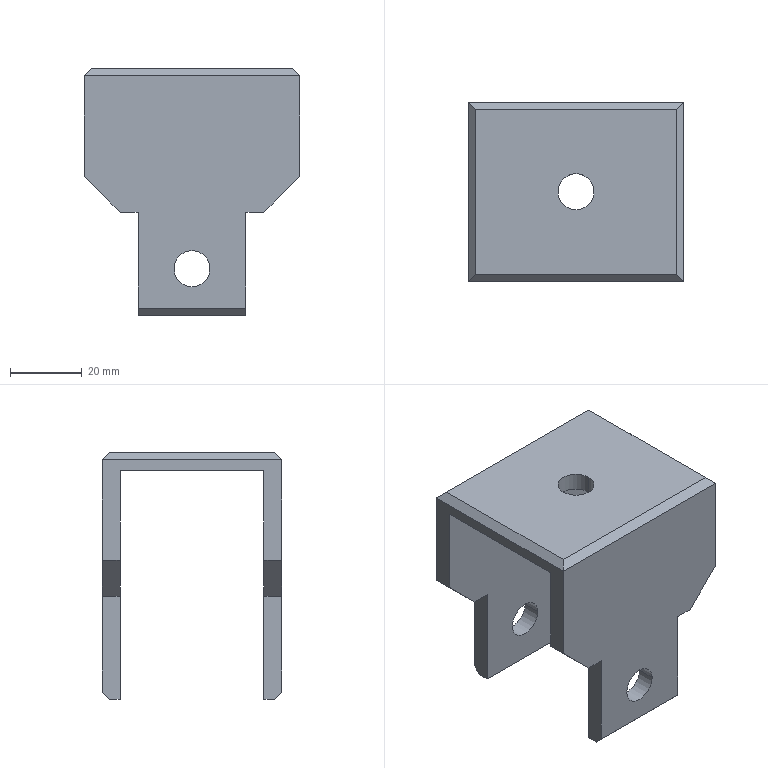Component | SolidWorks | AssemblyVibratoryFeederChassis-1_AssemblyWheel-1_WheelBracket-1 | 1 solid | 34 faces | box 60 x 50 x 68.72 mm | volume 41889 mm3 | plane 28 | cylinder 6 | commonest cylinder face diameters 10 x6
build123d program:
from build123d import *

# Parameters (mm, degrees)
EXTRUDE1_DEPTH = 60
SKETCH5_R      = 5
SKETCH5_W      = 15
SKETCH5_H      = 28.722
EXTRUDE2_DEPTH = 601.726
CHAMFER1_SIZE  = 10
SKETCH6_R      = 5
EXTRUDE3_DEPTH = 956.718
CHAMFER2_SIZE  = 2


with BuildPart() as part:
    # Sketch4 → Extrude1 (new body)
    with BuildSketch(Plane.XY):
        Polygon((-951.354, -526.906), (-901.354, -526.906), (-901.354, -595.627), (-906.354, -595.627), (-906.354, -531.906), (-946.354, -531.906), (-946.354, -595.627), (-951.354, -595.627), align=None)
    extrude(amount=-EXTRUDE1_DEPTH)

    # Sketch5 → Extrude2 (cut, through all)
    with BuildSketch(Plane.ZY.offset(951.354)):
        with Locations((-30, -582.627)):
            Circle(SKETCH5_R)
        with Locations((-52.5, -581.267)):
            Rectangle(SKETCH5_W, SKETCH5_H)
        with Locations((-7.5, -581.267)):
            Rectangle(SKETCH5_W, SKETCH5_H)
    extrude(amount=-EXTRUDE2_DEPTH, mode=Mode.SUBTRACT)

    # Chamfer1
    chamfer1_edges = [part.edges().sort_by_distance(p)[0] for p in [
        (-948.854, -566.906, -60),
        (-903.854, -566.906, -60),
        (-948.854, -566.906, 0),
        (-903.854, -566.906, 0),
    ]]
    chamfer(chamfer1_edges, length=CHAMFER1_SIZE)

    # Sketch6 → Extrude3 (cut, through all)
    with BuildSketch(Plane(origin=(0, -526.906, 0), x_dir=(1, 0, 0), z_dir=(0, 1, 0))):
        with Locations(Location((-926.354, 30, 0), (0, 0, 270))):
            Circle(SKETCH6_R)
    extrude(amount=-EXTRUDE3_DEPTH, mode=Mode.SUBTRACT)

    # Chamfer2
    chamfer2_edges = [part.edges().sort_by_distance(p)[0] for p in [
        (-951.354, -526.906, -30),
        (-901.354, -526.906, -30),
        (-926.354, -526.906, -60),
        (-951.354, -595.627, -30),
        (-901.354, -595.627, -30),
        (-926.354, -526.906, 0),
    ]]
    chamfer(chamfer2_edges, length=CHAMFER2_SIZE)


solid = part.part

# Placed as in the assembly
solid = solid.moved(Location((-307.449, -1207.53, 439.906), (90, -90, 0)))
STEP:
#1=COLOUR_RGB('',0.7922,0.8196,0.9333);
#2=FILL_AREA_STYLE_COLOUR('',#1);
#3=FILL_AREA_STYLE('',(#2));
#4=SURFACE_STYLE_FILL_AREA(#3);
#5=SURFACE_SIDE_STYLE('',(#4));
#6=SURFACE_STYLE_USAGE(.BOTH.,#5);
#7=PRESENTATION_STYLE_ASSIGNMENT((#6));
#8=CARTESIAN_POINT('',(-10.726,-11.07,-3.622));
#9=VERTEX_POINT('',#8);
#10=CARTESIAN_POINT('',(-11.12,-11.07,-3.622));
#11=VERTEX_POINT('',#10);
#12=CARTESIAN_POINT('',(-10.923,-11.07,-3.622));
#13=DIRECTION('',(-0.,-0.,-1.));
#14=DIRECTION('',(-1.,0.,0.));
#15=AXIS2_PLACEMENT_3D('',#12,#13,#14);
#16=CIRCLE('',#15,0.1969);
#17=EDGE_CURVE('',#9,#11,#16,.T.);
#18=ORIENTED_EDGE('',*,*,#17,.T.);
#19=CARTESIAN_POINT('',(-11.12,-11.07,-3.425));
#20=VERTEX_POINT('',#19);
#21=CARTESIAN_POINT('',(-11.12,-11.07,-6.131));
#22=DIRECTION('',(0.,0.,1.));
#23=VECTOR('',#22,39.37);
#24=LINE('',#21,#23);
#25=EDGE_CURVE('',#11,#20,#24,.T.);
#26=ORIENTED_EDGE('',*,*,#25,.T.);
#27=CARTESIAN_POINT('',(-10.726,-11.07,-3.425));
#28=VERTEX_POINT('',#27);
#29=CARTESIAN_POINT('',(-10.923,-11.07,-3.425));
#30=DIRECTION('',(0.,0.,1.));
#31=DIRECTION('',(1.,0.,0.));
#32=AXIS2_PLACEMENT_3D('',#29,#30,#31);
#33=CIRCLE('',#32,0.1969);
#34=EDGE_CURVE('',#20,#28,#33,.T.);
#35=ORIENTED_EDGE('',*,*,#34,.T.);
#36=CARTESIAN_POINT('',(-10.726,-11.07,-6.131));
#37=DIRECTION('',(0.,0.,1.));
#38=VECTOR('',#37,39.37);
#39=LINE('',#36,#38);
#40=EDGE_CURVE('',#9,#28,#39,.T.);
#41=ORIENTED_EDGE('',*,*,#40,.F.);
#42=EDGE_LOOP('',(#18,#26,#35,#41));
#43=FACE_OUTER_BOUND('',#42,.T.);
#44=CARTESIAN_POINT('',(-10.923,-11.07,-6.131));
#45=DIRECTION('',(0.,0.,1.));
#46=DIRECTION('',(1.,0.,0.));
#47=AXIS2_PLACEMENT_3D('',#44,#45,#46);
#48=CYLINDRICAL_SURFACE('',#47,0.1969);
#49=ADVANCED_FACE('',(#43),#48,.F.);
#50=CARTESIAN_POINT('',(-11.12,-10.086,-5.619));
#51=VERTEX_POINT('',#50);
#52=CARTESIAN_POINT('',(-10.726,-10.086,-5.619));
#53=VERTEX_POINT('',#52);
#54=CARTESIAN_POINT('',(-10.923,-10.086,-5.619));
#55=DIRECTION('',(-0.,-1.,0.));
#56=DIRECTION('',(1.,0.,0.));
#57=AXIS2_PLACEMENT_3D('',#54,#55,#56);
#58=CIRCLE('',#57,0.1969);
#59=EDGE_CURVE('',#51,#53,#58,.T.);
#60=ORIENTED_EDGE('',*,*,#59,.F.);
#61=CARTESIAN_POINT('',(-11.12,-10.283,-5.619));
#62=VERTEX_POINT('',#61);
#63=CARTESIAN_POINT('',(-11.12,-10.086,-5.619));
#64=DIRECTION('',(-0.,-1.,0.));
#65=VECTOR('',#64,39.37);
#66=LINE('',#63,#65);
#67=EDGE_CURVE('',#51,#62,#66,.T.);
#68=ORIENTED_EDGE('',*,*,#67,.T.);
#69=CARTESIAN_POINT('',(-10.726,-10.283,-5.619));
#70=VERTEX_POINT('',#69);
#71=CARTESIAN_POINT('',(-10.923,-10.283,-5.619));
#72=DIRECTION('',(-0.,-1.,0.));
#73=DIRECTION('',(1.,0.,0.));
#74=AXIS2_PLACEMENT_3D('',#71,#72,#73);
#75=CIRCLE('',#74,0.1969);
#76=EDGE_CURVE('',#62,#70,#75,.T.);
#77=ORIENTED_EDGE('',*,*,#76,.T.);
#78=CARTESIAN_POINT('',(-10.726,-10.086,-5.619));
#79=DIRECTION('',(-0.,-1.,0.));
#80=VECTOR('',#79,39.37);
#81=LINE('',#78,#80);
#82=EDGE_CURVE('',#53,#70,#81,.T.);
#83=ORIENTED_EDGE('',*,*,#82,.F.);
#84=EDGE_LOOP('',(#60,#68,#77,#83));
#85=FACE_OUTER_BOUND('',#84,.T.);
#86=CARTESIAN_POINT('',(-10.923,-10.086,-5.619));
#87=DIRECTION('',(-0.,-1.,0.));
#88=DIRECTION('',(1.,0.,0.));
#89=AXIS2_PLACEMENT_3D('',#86,#87,#88);
#90=CYLINDRICAL_SURFACE('',#89,0.1969);
#91=ADVANCED_FACE('',(#85),#90,.F.);
#92=CARTESIAN_POINT('',(-10.726,-11.857,-5.619));
#93=VERTEX_POINT('',#92);
#94=CARTESIAN_POINT('',(-11.12,-11.857,-5.619));
#95=VERTEX_POINT('',#94);
#96=CARTESIAN_POINT('',(-10.923,-11.857,-5.619));
#97=DIRECTION('',(0.,1.,-0.));
#98=DIRECTION('',(-1.,0.,0.));
#99=AXIS2_PLACEMENT_3D('',#96,#97,#98);
#100=CIRCLE('',#99,0.1969);
#101=EDGE_CURVE('',#93,#95,#100,.T.);
#102=ORIENTED_EDGE('',*,*,#101,.T.);
#103=CARTESIAN_POINT('',(-11.12,-12.054,-5.619));
#104=VERTEX_POINT('',#103);
#105=CARTESIAN_POINT('',(-11.12,-10.086,-5.619));
#106=DIRECTION('',(-0.,-1.,0.));
#107=VECTOR('',#106,39.37);
#108=LINE('',#105,#107);
#109=EDGE_CURVE('',#95,#104,#108,.T.);
#110=ORIENTED_EDGE('',*,*,#109,.T.);
#111=CARTESIAN_POINT('',(-10.726,-12.054,-5.619));
#112=VERTEX_POINT('',#111);
#113=CARTESIAN_POINT('',(-10.923,-12.054,-5.619));
#114=DIRECTION('',(-0.,-1.,0.));
#115=DIRECTION('',(1.,0.,0.));
#116=AXIS2_PLACEMENT_3D('',#113,#114,#115);
#117=CIRCLE('',#116,0.1969);
#118=EDGE_CURVE('',#104,#112,#117,.T.);
#119=ORIENTED_EDGE('',*,*,#118,.T.);
#120=CARTESIAN_POINT('',(-10.726,-10.086,-5.619));
#121=DIRECTION('',(-0.,-1.,0.));
#122=VECTOR('',#121,39.37);
#123=LINE('',#120,#122);
#124=EDGE_CURVE('',#93,#112,#123,.T.);
#125=ORIENTED_EDGE('',*,*,#124,.F.);
#126=EDGE_LOOP('',(#102,#110,#119,#125));
#127=FACE_OUTER_BOUND('',#126,.T.);
#128=CARTESIAN_POINT('',(-10.923,-10.086,-5.619));
#129=DIRECTION('',(-0.,-1.,0.));
#130=DIRECTION('',(1.,0.,0.));
#131=AXIS2_PLACEMENT_3D('',#128,#129,#130);
#132=CYLINDRICAL_SURFACE('',#131,0.1969);
#133=ADVANCED_FACE('',(#127),#132,.F.);
#134=CARTESIAN_POINT('',(-10.923,-12.054,-5.619));
#135=DIRECTION('',(-0.,-1.,0.));
#136=DIRECTION('',(1.,0.,0.));
#137=AXIS2_PLACEMENT_3D('',#134,#135,#136);
#138=CIRCLE('',#137,0.1969);
#139=EDGE_CURVE('',#112,#104,#138,.T.);
#140=ORIENTED_EDGE('',*,*,#139,.F.);
#141=ORIENTED_EDGE('',*,*,#118,.F.);
#142=EDGE_LOOP('',(#140,#141));
#143=FACE_BOUND('',#142,.T.);
#144=CARTESIAN_POINT('',(-11.514,-12.054,-6.052));
#145=VERTEX_POINT('',#144);
#146=CARTESIAN_POINT('',(-11.514,-12.054,-5.));
#147=VERTEX_POINT('',#146);
#148=CARTESIAN_POINT('',(-11.514,-12.054,-5.));
#149=DIRECTION('',(-0.,0.,1.));
#150=VECTOR('',#149,39.37);
#151=LINE('',#148,#150);
#152=EDGE_CURVE('',#145,#147,#151,.T.);
#153=ORIENTED_EDGE('',*,*,#152,.F.);
#154=CARTESIAN_POINT('',(-10.333,-12.054,-6.052));
#155=VERTEX_POINT('',#154);
#156=CARTESIAN_POINT('',(-12.104,-12.054,-6.052));
#157=DIRECTION('',(1.,-0.,-0.));
#158=VECTOR('',#157,39.37);
#159=LINE('',#156,#158);
#160=EDGE_CURVE('',#145,#155,#159,.T.);
#161=ORIENTED_EDGE('',*,*,#160,.T.);
#162=CARTESIAN_POINT('',(-10.333,-12.054,-5.));
#163=VERTEX_POINT('',#162);
#164=CARTESIAN_POINT('',(-10.333,-12.054,-5.));
#165=DIRECTION('',(-0.,-0.,-1.));
#166=VECTOR('',#165,39.37);
#167=LINE('',#164,#166);
#168=EDGE_CURVE('',#163,#155,#167,.T.);
#169=ORIENTED_EDGE('',*,*,#168,.F.);
#170=CARTESIAN_POINT('',(-10.136,-12.054,-5.));
#171=VERTEX_POINT('',#170);
#172=CARTESIAN_POINT('',(-10.333,-12.054,-5.));
#173=DIRECTION('',(-1.,0.,0.));
#174=VECTOR('',#173,39.37);
#175=LINE('',#172,#174);
#176=EDGE_CURVE('',#171,#163,#175,.T.);
#177=ORIENTED_EDGE('',*,*,#176,.F.);
#178=CARTESIAN_POINT('',(-9.742,-12.054,-4.606));
#179=VERTEX_POINT('',#178);
#180=CARTESIAN_POINT('',(-10.333,-12.054,-5.197));
#181=DIRECTION('',(0.7071,0.,0.7071));
#182=VECTOR('',#181,39.37);
#183=LINE('',#180,#182);
#184=EDGE_CURVE('',#171,#179,#183,.T.);
#185=ORIENTED_EDGE('',*,*,#184,.T.);
#186=CARTESIAN_POINT('',(-9.742,-12.054,-3.504));
#187=VERTEX_POINT('',#186);
#188=CARTESIAN_POINT('',(-9.742,-12.054,-3.425));
#189=DIRECTION('',(-0.,-0.,-1.));
#190=VECTOR('',#189,39.37);
#191=LINE('',#188,#190);
#192=EDGE_CURVE('',#187,#179,#191,.T.);
#193=ORIENTED_EDGE('',*,*,#192,.F.);
#194=CARTESIAN_POINT('',(-12.104,-12.054,-3.504));
#195=VERTEX_POINT('',#194);
#196=CARTESIAN_POINT('',(-12.104,-12.054,-3.504));
#197=DIRECTION('',(-1.,0.,0.));
#198=VECTOR('',#197,39.37);
#199=LINE('',#196,#198);
#200=EDGE_CURVE('',#187,#195,#199,.T.);
#201=ORIENTED_EDGE('',*,*,#200,.T.);
#202=CARTESIAN_POINT('',(-12.104,-12.054,-4.606));
#203=VERTEX_POINT('',#202);
#204=CARTESIAN_POINT('',(-12.104,-12.054,-3.425));
#205=DIRECTION('',(-0.,-0.,-1.));
#206=VECTOR('',#205,39.37);
#207=LINE('',#204,#206);
#208=EDGE_CURVE('',#195,#203,#207,.T.);
#209=ORIENTED_EDGE('',*,*,#208,.T.);
#210=CARTESIAN_POINT('',(-11.711,-12.054,-5.));
#211=VERTEX_POINT('',#210);
#212=CARTESIAN_POINT('',(-12.695,-12.054,-4.016));
#213=DIRECTION('',(0.7071,-0.,-0.7071));
#214=VECTOR('',#213,39.37);
#215=LINE('',#212,#214);
#216=EDGE_CURVE('',#203,#211,#215,.T.);
#217=ORIENTED_EDGE('',*,*,#216,.T.);
#218=CARTESIAN_POINT('',(-11.514,-12.054,-5.));
#219=DIRECTION('',(-1.,0.,0.));
#220=VECTOR('',#219,39.37);
#221=LINE('',#218,#220);
#222=EDGE_CURVE('',#147,#211,#221,.T.);
#223=ORIENTED_EDGE('',*,*,#222,.F.);
#224=EDGE_LOOP('',(#153,#161,#169,#177,#185,#193,#201,#209,#217,#223));
#225=FACE_OUTER_BOUND('',#224,.T.);
#226=CARTESIAN_POINT('',(-12.104,-12.054,-3.425));
#227=DIRECTION('',(-0.,-1.,0.));
#228=DIRECTION('',(1.,-0.,-0.));
#229=AXIS2_PLACEMENT_3D('',#226,#227,#228);
#230=PLANE('',#229);
#231=ADVANCED_FACE('',(#143,#225),#230,.T.);
#232=CARTESIAN_POINT('',(-9.821,-11.975,-3.425));
#233=VERTEX_POINT('',#232);
#234=CARTESIAN_POINT('',(-9.821,-10.164,-3.425));
#235=VERTEX_POINT('',#234);
#236=CARTESIAN_POINT('',(-9.821,-10.086,-3.425));
#237=DIRECTION('',(0.,1.,-0.));
#238=VECTOR('',#237,39.37);
#239=LINE('',#236,#238);
#240=EDGE_CURVE('',#233,#235,#239,.T.);
#241=ORIENTED_EDGE('',*,*,#240,.T.);
#242=CARTESIAN_POINT('',(-12.026,-10.164,-3.425));
#243=VERTEX_POINT('',#242);
#244=CARTESIAN_POINT('',(-12.104,-10.164,-3.425));
#245=DIRECTION('',(-1.,0.,0.));
#246=VECTOR('',#245,39.37);
#247=LINE('',#244,#246);
#248=EDGE_CURVE('',#235,#243,#247,.T.);
#249=ORIENTED_EDGE('',*,*,#248,.T.);
#250=CARTESIAN_POINT('',(-12.026,-11.975,-3.425));
#251=VERTEX_POINT('',#250);
#252=CARTESIAN_POINT('',(-12.026,-12.054,-3.425));
#253=DIRECTION('',(-0.,-1.,0.));
#254=VECTOR('',#253,39.37);
#255=LINE('',#252,#254);
#256=EDGE_CURVE('',#243,#251,#255,.T.);
#257=ORIENTED_EDGE('',*,*,#256,.T.);
#258=CARTESIAN_POINT('',(-12.104,-11.975,-3.425));
#259=DIRECTION('',(1.,-0.,-0.));
#260=VECTOR('',#259,39.37);
#261=LINE('',#258,#260);
#262=EDGE_CURVE('',#251,#233,#261,.T.);
#263=ORIENTED_EDGE('',*,*,#262,.T.);
#264=EDGE_LOOP('',(#241,#249,#257,#263));
#265=FACE_OUTER_BOUND('',#264,.T.);
#266=CARTESIAN_POINT('',(-10.923,-11.07,-3.425));
#267=DIRECTION('',(0.,0.,1.));
#268=DIRECTION('',(1.,0.,0.));
#269=AXIS2_PLACEMENT_3D('',#266,#267,#268);
#270=CIRCLE('',#269,0.1969);
#271=EDGE_CURVE('',#28,#20,#270,.T.);
#272=ORIENTED_EDGE('',*,*,#271,.F.);
#273=ORIENTED_EDGE('',*,*,#34,.F.);
#274=EDGE_LOOP('',(#272,#273));
#275=FACE_BOUND('',#274,.T.);
#276=CARTESIAN_POINT('',(-12.104,-12.054,-3.425));
#277=DIRECTION('',(0.,0.,1.));
#278=DIRECTION('',(1.,-0.,-0.));
#279=AXIS2_PLACEMENT_3D('',#276,#277,#278);
#280=PLANE('',#279);
#281=ADVANCED_FACE('',(#265,#275),#280,.T.);
#282=CARTESIAN_POINT('',(-10.923,-10.086,-5.619));
#283=DIRECTION('',(-0.,-1.,0.));
#284=DIRECTION('',(1.,0.,0.));
#285=AXIS2_PLACEMENT_3D('',#282,#283,#284);
#286=CIRCLE('',#285,0.1969);
#287=EDGE_CURVE('',#53,#51,#286,.T.);
#288=ORIENTED_EDGE('',*,*,#287,.T.);
#289=ORIENTED_EDGE('',*,*,#59,.T.);
#290=EDGE_LOOP('',(#288,#289));
#291=FACE_BOUND('',#290,.T.);
#292=CARTESIAN_POINT('',(-10.333,-10.086,-5.));
#293=VERTEX_POINT('',#292);
#294=CARTESIAN_POINT('',(-10.333,-10.086,-6.052));
#295=VERTEX_POINT('',#294);
#296=CARTESIAN_POINT('',(-10.333,-10.086,-5.));
#297=DIRECTION('',(-0.,-0.,-1.));
#298=VECTOR('',#297,39.37);
#299=LINE('',#296,#298);
#300=EDGE_CURVE('',#293,#295,#299,.T.);
#301=ORIENTED_EDGE('',*,*,#300,.T.);
#302=CARTESIAN_POINT('',(-11.514,-10.086,-6.052));
#303=VERTEX_POINT('',#302);
#304=CARTESIAN_POINT('',(-12.104,-10.086,-6.052));
#305=DIRECTION('',(-1.,0.,0.));
#306=VECTOR('',#305,39.37);
#307=LINE('',#304,#306);
#308=EDGE_CURVE('',#295,#303,#307,.T.);
#309=ORIENTED_EDGE('',*,*,#308,.T.);
#310=CARTESIAN_POINT('',(-11.514,-10.086,-5.));
#311=VERTEX_POINT('',#310);
#312=CARTESIAN_POINT('',(-11.514,-10.086,-5.));
#313=DIRECTION('',(-0.,0.,1.));
#314=VECTOR('',#313,39.37);
#315=LINE('',#312,#314);
#316=EDGE_CURVE('',#303,#311,#315,.T.);
#317=ORIENTED_EDGE('',*,*,#316,.T.);
#318=CARTESIAN_POINT('',(-11.711,-10.086,-5.));
#319=VERTEX_POINT('',#318);
#320=CARTESIAN_POINT('',(-11.514,-10.086,-5.));
#321=DIRECTION('',(-1.,0.,0.));
#322=VECTOR('',#321,39.37);
#323=LINE('',#320,#322);
#324=EDGE_CURVE('',#311,#319,#323,.T.);
#325=ORIENTED_EDGE('',*,*,#324,.T.);
#326=CARTESIAN_POINT('',(-12.104,-10.086,-4.606));
#327=VERTEX_POINT('',#326);
#328=CARTESIAN_POINT('',(-12.695,-10.086,-4.016));
#329=DIRECTION('',(-0.7071,0.,0.7071));
#330=VECTOR('',#329,39.37);
#331=LINE('',#328,#330);
#332=EDGE_CURVE('',#319,#327,#331,.T.);
#333=ORIENTED_EDGE('',*,*,#332,.T.);
#334=CARTESIAN_POINT('',(-12.104,-10.086,-3.504));
#335=VERTEX_POINT('',#334);
#336=CARTESIAN_POINT('',(-12.104,-10.086,-3.425));
#337=DIRECTION('',(0.,0.,1.));
#338=VECTOR('',#337,39.37);
#339=LINE('',#336,#338);
#340=EDGE_CURVE('',#327,#335,#339,.T.);
#341=ORIENTED_EDGE('',*,*,#340,.T.);
#342=CARTESIAN_POINT('',(-9.742,-10.086,-3.504));
#343=VERTEX_POINT('',#342);
#344=CARTESIAN_POINT('',(-12.104,-10.086,-3.504));
#345=DIRECTION('',(1.,-0.,-0.));
#346=VECTOR('',#345,39.37);
#347=LINE('',#344,#346);
#348=EDGE_CURVE('',#335,#343,#347,.T.);
#349=ORIENTED_EDGE('',*,*,#348,.T.);
#350=CARTESIAN_POINT('',(-9.742,-10.086,-4.606));
#351=VERTEX_POINT('',#350);
#352=CARTESIAN_POINT('',(-9.742,-10.086,-3.425));
#353=DIRECTION('',(0.,0.,1.));
#354=VECTOR('',#353,39.37);
#355=LINE('',#352,#354);
#356=EDGE_CURVE('',#351,#343,#355,.T.);
#357=ORIENTED_EDGE('',*,*,#356,.F.);
#358=CARTESIAN_POINT('',(-10.136,-10.086,-5.));
#359=VERTEX_POINT('',#358);
#360=CARTESIAN_POINT('',(-10.333,-10.086,-5.197));
#361=DIRECTION('',(-0.7071,-0.,-0.7071));
#362=VECTOR('',#361,39.37);
#363=LINE('',#360,#362);
#364=EDGE_CURVE('',#351,#359,#363,.T.);
#365=ORIENTED_EDGE('',*,*,#364,.T.);
#366=CARTESIAN_POINT('',(-10.333,-10.086,-5.));
#367=DIRECTION('',(-1.,0.,0.));
#368=VECTOR('',#367,39.37);
#369=LINE('',#366,#368);
#370=EDGE_CURVE('',#359,#293,#369,.T.);
#371=ORIENTED_EDGE('',*,*,#370,.T.);
#372=EDGE_LOOP('',(#301,#309,#317,#325,#333,#341,#349,#357,#365,#371));
#373=FACE_OUTER_BOUND('',#372,.T.);
#374=CARTESIAN_POINT('',(-12.104,-10.086,-3.425));
#375=DIRECTION('',(0.,1.,-0.));
#376=DIRECTION('',(-1.,0.,0.));
#377=AXIS2_PLACEMENT_3D('',#374,#375,#376);
#378=PLANE('',#377);
#379=ADVANCED_FACE('',(#291,#373),#378,.T.);
#380=CARTESIAN_POINT('',(-11.514,-10.164,-6.131));
#381=VERTEX_POINT('',#380);
#382=CARTESIAN_POINT('',(-11.514,-10.283,-6.131));
#383=VERTEX_POINT('',#382);
#384=CARTESIAN_POINT('',(-11.514,-10.086,-6.131));
#385=DIRECTION('',(-0.,-1.,0.));
#386=VECTOR('',#385,39.37);
#387=LINE('',#384,#386);
#388=EDGE_CURVE('',#381,#383,#387,.T.);
#389=ORIENTED_EDGE('',*,*,#388,.F.);
#390=CARTESIAN_POINT('',(-10.333,-10.164,-6.131));
#391=VERTEX_POINT('',#390);
#392=CARTESIAN_POINT('',(-12.104,-10.164,-6.131));
#393=DIRECTION('',(1.,-0.,-0.));
#394=VECTOR('',#393,39.37);
#395=LINE('',#392,#394);
#396=EDGE_CURVE('',#381,#391,#395,.T.);
#397=ORIENTED_EDGE('',*,*,#396,.T.);
#398=CARTESIAN_POINT('',(-10.333,-10.283,-6.131));
#399=VERTEX_POINT('',#398);
#400=CARTESIAN_POINT('',(-10.333,-10.086,-6.131));
#401=DIRECTION('',(-0.,-1.,0.));
#402=VECTOR('',#401,39.37);
#403=LINE('',#400,#402);
#404=EDGE_CURVE('',#391,#399,#403,.T.);
#405=ORIENTED_EDGE('',*,*,#404,.T.);
#406=CARTESIAN_POINT('',(-12.104,-10.283,-6.131));
#407=DIRECTION('',(1.,-0.,-0.));
#408=VECTOR('',#407,39.37);
#409=LINE('',#406,#408);
#410=EDGE_CURVE('',#383,#399,#409,.T.);
#411=ORIENTED_EDGE('',*,*,#410,.F.);
#412=EDGE_LOOP('',(#389,#397,#405,#411));
#413=FACE_OUTER_BOUND('',#412,.T.);
#414=CARTESIAN_POINT('',(-12.104,-10.086,-6.131));
#415=DIRECTION('',(-0.,-0.,-1.));
#416=DIRECTION('',(-1.,0.,0.));
#417=AXIS2_PLACEMENT_3D('',#414,#415,#416);
#418=PLANE('',#417);
#419=ADVANCED_FACE('',(#413),#418,.T.);
#420=CARTESIAN_POINT('',(-10.923,-10.283,-5.619));
#421=DIRECTION('',(-0.,-1.,0.));
#422=DIRECTION('',(1.,0.,0.));
#423=AXIS2_PLACEMENT_3D('',#420,#421,#422);
#424=CIRCLE('',#423,0.1969);
#425=EDGE_CURVE('',#70,#62,#424,.T.);
#426=ORIENTED_EDGE('',*,*,#425,.F.);
#427=ORIENTED_EDGE('',*,*,#76,.F.);
#428=EDGE_LOOP('',(#426,#427));
#429=FACE_BOUND('',#428,.T.);
#430=CARTESIAN_POINT('',(-10.136,-10.283,-5.));
#431=VERTEX_POINT('',#430);
#432=CARTESIAN_POINT('',(-10.333,-10.283,-5.));
#433=VERTEX_POINT('',#432);
#434=CARTESIAN_POINT('',(-12.104,-10.283,-5.));
#435=DIRECTION('',(-1.,0.,0.));
#436=VECTOR('',#435,39.37);
#437=LINE('',#434,#436);
#438=EDGE_CURVE('',#431,#433,#437,.T.);
#439=ORIENTED_EDGE('',*,*,#438,.F.);
#440=CARTESIAN_POINT('',(-9.742,-10.283,-4.606));
#441=VERTEX_POINT('',#440);
#442=CARTESIAN_POINT('',(-10.431,-10.283,-5.295));
#443=DIRECTION('',(0.7071,0.,0.7071));
#444=VECTOR('',#443,39.37);
#445=LINE('',#442,#444);
#446=EDGE_CURVE('',#431,#441,#445,.T.);
#447=ORIENTED_EDGE('',*,*,#446,.T.);
#448=CARTESIAN_POINT('',(-9.742,-10.283,-3.622));
#449=VERTEX_POINT('',#448);
#450=CARTESIAN_POINT('',(-9.742,-10.283,-3.622));
#451=DIRECTION('',(-0.,-0.,-1.));
#452=VECTOR('',#451,39.37);
#453=LINE('',#450,#452);
#454=EDGE_CURVE('',#449,#441,#453,.T.);
#455=ORIENTED_EDGE('',*,*,#454,.F.);
#456=CARTESIAN_POINT('',(-12.104,-10.283,-3.622));
#457=VERTEX_POINT('',#456);
#458=CARTESIAN_POINT('',(-12.104,-10.283,-3.622));
#459=DIRECTION('',(1.,-0.,-0.));
#460=VECTOR('',#459,39.37);
#461=LINE('',#458,#460);
#462=EDGE_CURVE('',#457,#449,#461,.T.);
#463=ORIENTED_EDGE('',*,*,#462,.F.);
#464=CARTESIAN_POINT('',(-12.104,-10.283,-4.606));
#465=VERTEX_POINT('',#464);
#466=CARTESIAN_POINT('',(-12.104,-10.283,-3.622));
#467=DIRECTION('',(-0.,-0.,-1.));
#468=VECTOR('',#467,39.37);
#469=LINE('',#466,#468);
#470=EDGE_CURVE('',#457,#465,#469,.T.);
#471=ORIENTED_EDGE('',*,*,#470,.T.);
#472=CARTESIAN_POINT('',(-11.711,-10.283,-5.));
#473=VERTEX_POINT('',#472);
#474=CARTESIAN_POINT('',(-12.596,-10.283,-4.114));
#475=DIRECTION('',(0.7071,-0.,-0.7071));
#476=VECTOR('',#475,39.37);
#477=LINE('',#474,#476);
#478=EDGE_CURVE('',#465,#473,#477,.T.);
#479=ORIENTED_EDGE('',*,*,#478,.T.);
#480=CARTESIAN_POINT('',(-11.514,-10.283,-5.));
#481=VERTEX_POINT('',#480);
#482=CARTESIAN_POINT('',(-12.104,-10.283,-5.));
#483=DIRECTION('',(-1.,0.,0.));
#484=VECTOR('',#483,39.37);
#485=LINE('',#482,#484);
#486=EDGE_CURVE('',#481,#473,#485,.T.);
#487=ORIENTED_EDGE('',*,*,#486,.F.);
#488=CARTESIAN_POINT('',(-11.514,-10.283,-3.622));
#489=DIRECTION('',(-0.,0.,1.));
#490=VECTOR('',#489,39.37);
#491=LINE('',#488,#490);
#492=EDGE_CURVE('',#383,#481,#491,.T.);
#493=ORIENTED_EDGE('',*,*,#492,.F.);
#494=ORIENTED_EDGE('',*,*,#410,.T.);
#495=CARTESIAN_POINT('',(-10.333,-10.283,-3.622));
#496=DIRECTION('',(-0.,-0.,-1.));
#497=VECTOR('',#496,39.37);
#498=LINE('',#495,#497);
#499=EDGE_CURVE('',#433,#399,#498,.T.);
#500=ORIENTED_EDGE('',*,*,#499,.F.);
#501=EDGE_LOOP('',(#439,#447,#455,#463,#471,#479,#487,#493,#494,#500));
#502=FACE_OUTER_BOUND('',#501,.T.);
#503=CARTESIAN_POINT('',(-12.104,-10.283,-3.622));
#504=DIRECTION('',(-0.,-1.,0.));
#505=DIRECTION('',(1.,-0.,-0.));
#506=AXIS2_PLACEMENT_3D('',#503,#504,#505);
#507=PLANE('',#506);
#508=ADVANCED_FACE('',(#429,#502),#507,.T.);
#509=ORIENTED_EDGE('',*,*,#17,.F.);
#510=CARTESIAN_POINT('',(-10.923,-11.07,-3.622));
#511=DIRECTION('',(-0.,-0.,-1.));
#512=DIRECTION('',(-1.,0.,0.));
#513=AXIS2_PLACEMENT_3D('',#510,#511,#512);
#514=CIRCLE('',#513,0.1969);
#515=EDGE_CURVE('',#11,#9,#514,.T.);
#516=ORIENTED_EDGE('',*,*,#515,.F.);
#517=EDGE_LOOP('',(#509,#516));
#518=FACE_BOUND('',#517,.T.);
#519=CARTESIAN_POINT('',(-9.742,-11.857,-3.622));
#520=VERTEX_POINT('',#519);
#521=CARTESIAN_POINT('',(-9.742,-11.857,-3.622));
#522=DIRECTION('',(0.,1.,-0.));
#523=VECTOR('',#522,39.37);
#524=LINE('',#521,#523);
#525=EDGE_CURVE('',#520,#449,#524,.T.);
#526=ORIENTED_EDGE('',*,*,#525,.F.);
#527=CARTESIAN_POINT('',(-12.104,-11.857,-3.622));
#528=VERTEX_POINT('',#527);
#529=CARTESIAN_POINT('',(-12.104,-11.857,-3.622));
#530=DIRECTION('',(1.,-0.,-0.));
#531=VECTOR('',#530,39.37);
#532=LINE('',#529,#531);
#533=EDGE_CURVE('',#528,#520,#532,.T.);
#534=ORIENTED_EDGE('',*,*,#533,.F.);
#535=CARTESIAN_POINT('',(-12.104,-11.857,-3.622));
#536=DIRECTION('',(0.,1.,-0.));
#537=VECTOR('',#536,39.37);
#538=LINE('',#535,#537);
#539=EDGE_CURVE('',#528,#457,#538,.T.);
#540=ORIENTED_EDGE('',*,*,#539,.T.);
#541=ORIENTED_EDGE('',*,*,#462,.T.);
#542=EDGE_LOOP('',(#526,#534,#540,#541));
#543=FACE_OUTER_BOUND('',#542,.T.);
#544=CARTESIAN_POINT('',(-12.104,-11.857,-3.622));
#545=DIRECTION('',(-0.,-0.,-1.));
#546=DIRECTION('',(-1.,0.,0.));
#547=AXIS2_PLACEMENT_3D('',#544,#545,#546);
#548=PLANE('',#547);
#549=ADVANCED_FACE('',(#518,#543),#548,.T.);
#550=ORIENTED_EDGE('',*,*,#101,.F.);
#551=CARTESIAN_POINT('',(-10.923,-11.857,-5.619));
#552=DIRECTION('',(0.,1.,-0.));
#553=DIRECTION('',(-1.,0.,0.));
#554=AXIS2_PLACEMENT_3D('',#551,#552,#553);
#555=CIRCLE('',#554,0.1969);
#556=EDGE_CURVE('',#95,#93,#555,.T.);
#557=ORIENTED_EDGE('',*,*,#556,.F.);
#558=EDGE_LOOP('',(#550,#557));
#559=FACE_BOUND('',#558,.T.);
#560=CARTESIAN_POINT('',(-9.742,-11.857,-4.606));
#561=VERTEX_POINT('',#560);
#562=CARTESIAN_POINT('',(-9.742,-11.857,-3.622));
#563=DIRECTION('',(0.,0.,1.));
#564=VECTOR('',#563,39.37);
#565=LINE('',#562,#564);
#566=EDGE_CURVE('',#561,#520,#565,.T.);
#567=ORIENTED_EDGE('',*,*,#566,.F.);
#568=CARTESIAN_POINT('',(-10.136,-11.857,-5.));
#569=VERTEX_POINT('',#568);
#570=CARTESIAN_POINT('',(-10.431,-11.857,-5.295));
#571=DIRECTION('',(-0.7071,-0.,-0.7071));
#572=VECTOR('',#571,39.37);
#573=LINE('',#570,#572);
#574=EDGE_CURVE('',#561,#569,#573,.T.);
#575=ORIENTED_EDGE('',*,*,#574,.T.);
#576=CARTESIAN_POINT('',(-10.333,-11.857,-5.));
#577=VERTEX_POINT('',#576);
#578=CARTESIAN_POINT('',(-12.104,-11.857,-5.));
#579=DIRECTION('',(1.,-0.,-0.));
#580=VECTOR('',#579,39.37);
#581=LINE('',#578,#580);
#582=EDGE_CURVE('',#577,#569,#581,.T.);
#583=ORIENTED_EDGE('',*,*,#582,.F.);
#584=CARTESIAN_POINT('',(-10.333,-11.857,-6.131));
#585=VERTEX_POINT('',#584);
#586=CARTESIAN_POINT('',(-10.333,-11.857,-3.622));
#587=DIRECTION('',(0.,0.,1.));
#588=VECTOR('',#587,39.37);
#589=LINE('',#586,#588);
#590=EDGE_CURVE('',#585,#577,#589,.T.);
#591=ORIENTED_EDGE('',*,*,#590,.F.);
#592=CARTESIAN_POINT('',(-11.514,-11.857,-6.131));
#593=VERTEX_POINT('',#592);
#594=CARTESIAN_POINT('',(-12.104,-11.857,-6.131));
#595=DIRECTION('',(1.,-0.,-0.));
#596=VECTOR('',#595,39.37);
#597=LINE('',#594,#596);
#598=EDGE_CURVE('',#593,#585,#597,.T.);
#599=ORIENTED_EDGE('',*,*,#598,.F.);
#600=CARTESIAN_POINT('',(-11.514,-11.857,-5.));
#601=VERTEX_POINT('',#600);
#602=CARTESIAN_POINT('',(-11.514,-11.857,-3.622));
#603=DIRECTION('',(0.,-0.,-1.));
#604=VECTOR('',#603,39.37);
#605=LINE('',#602,#604);
#606=EDGE_CURVE('',#601,#593,#605,.T.);
#607=ORIENTED_EDGE('',*,*,#606,.F.);
#608=CARTESIAN_POINT('',(-11.711,-11.857,-5.));
#609=VERTEX_POINT('',#608);
#610=CARTESIAN_POINT('',(-12.104,-11.857,-5.));
#611=DIRECTION('',(1.,-0.,-0.));
#612=VECTOR('',#611,39.37);
#613=LINE('',#610,#612);
#614=EDGE_CURVE('',#609,#601,#613,.T.);
#615=ORIENTED_EDGE('',*,*,#614,.F.);
#616=CARTESIAN_POINT('',(-12.104,-11.857,-4.606));
#617=VERTEX_POINT('',#616);
#618=CARTESIAN_POINT('',(-12.596,-11.857,-4.114));
#619=DIRECTION('',(-0.7071,0.,0.7071));
#620=VECTOR('',#619,39.37);
#621=LINE('',#618,#620);
#622=EDGE_CURVE('',#609,#617,#621,.T.);
#623=ORIENTED_EDGE('',*,*,#622,.T.);
#624=CARTESIAN_POINT('',(-12.104,-11.857,-3.622));
#625=DIRECTION('',(0.,0.,1.));
#626=VECTOR('',#625,39.37);
#627=LINE('',#624,#626);
#628=EDGE_CURVE('',#617,#528,#627,.T.);
#629=ORIENTED_EDGE('',*,*,#628,.T.);
#630=ORIENTED_EDGE('',*,*,#533,.T.);
#631=EDGE_LOOP('',(#567,#575,#583,#591,#599,#607,#615,#623,#629,#630));
#632=FACE_OUTER_BOUND('',#631,.T.);
#633=CARTESIAN_POINT('',(-12.104,-11.857,-3.622));
#634=DIRECTION('',(0.,1.,-0.));
#635=DIRECTION('',(-1.,0.,0.));
#636=AXIS2_PLACEMENT_3D('',#633,#634,#635);
#637=PLANE('',#636);
#638=ADVANCED_FACE('',(#559,#632),#637,.T.);
#639=CARTESIAN_POINT('',(-10.333,-11.975,-6.131));
#640=VERTEX_POINT('',#639);
#641=CARTESIAN_POINT('',(-10.333,-10.086,-6.131));
#642=DIRECTION('',(-0.,-1.,0.));
#643=VECTOR('',#642,39.37);
#644=LINE('',#641,#643);
#645=EDGE_CURVE('',#585,#640,#644,.T.);
#646=ORIENTED_EDGE('',*,*,#645,.T.);
#647=CARTESIAN_POINT('',(-11.514,-11.975,-6.131));
#648=VERTEX_POINT('',#647);
#649=CARTESIAN_POINT('',(-12.104,-11.975,-6.131));
#650=DIRECTION('',(-1.,0.,0.));
#651=VECTOR('',#650,39.37);
#652=LINE('',#649,#651);
#653=EDGE_CURVE('',#640,#648,#652,.T.);
#654=ORIENTED_EDGE('',*,*,#653,.T.);
#655=CARTESIAN_POINT('',(-11.514,-10.086,-6.131));
#656=DIRECTION('',(-0.,-1.,0.));
#657=VECTOR('',#656,39.37);
#658=LINE('',#655,#657);
#659=EDGE_CURVE('',#593,#648,#658,.T.);
#660=ORIENTED_EDGE('',*,*,#659,.F.);
#661=ORIENTED_EDGE('',*,*,#598,.T.);
#662=EDGE_LOOP('',(#646,#654,#660,#661));
#663=FACE_OUTER_BOUND('',#662,.T.);
#664=CARTESIAN_POINT('',(-12.104,-11.857,-6.131));
#665=DIRECTION('',(-0.,-0.,-1.));
#666=DIRECTION('',(-1.,0.,0.));
#667=AXIS2_PLACEMENT_3D('',#664,#665,#666);
#668=PLANE('',#667);
#669=ADVANCED_FACE('',(#663),#668,.T.);
#670=ORIENTED_EDGE('',*,*,#208,.F.);
#671=CARTESIAN_POINT('',(-12.104,-12.054,-3.504));
#672=DIRECTION('',(0.,1.,-0.));
#673=VECTOR('',#672,39.37);
#674=LINE('',#671,#673);
#675=EDGE_CURVE('',#195,#335,#674,.T.);
#676=ORIENTED_EDGE('',*,*,#675,.T.);
#677=ORIENTED_EDGE('',*,*,#340,.F.);
#678=CARTESIAN_POINT('',(-12.104,-10.283,-4.606));
#679=DIRECTION('',(-0.,-1.,0.));
#680=VECTOR('',#679,39.37);
#681=LINE('',#678,#680);
#682=EDGE_CURVE('',#327,#465,#681,.T.);
#683=ORIENTED_EDGE('',*,*,#682,.T.);
#684=ORIENTED_EDGE('',*,*,#470,.F.);
#685=ORIENTED_EDGE('',*,*,#539,.F.);
#686=ORIENTED_EDGE('',*,*,#628,.F.);
#687=CARTESIAN_POINT('',(-12.104,-12.054,-4.606));
#688=DIRECTION('',(-0.,-1.,0.));
#689=VECTOR('',#688,39.37);
#690=LINE('',#687,#689);
#691=EDGE_CURVE('',#617,#203,#690,.T.);
#692=ORIENTED_EDGE('',*,*,#691,.T.);
#693=EDGE_LOOP('',(#670,#676,#677,#683,#684,#685,#686,#692));
#694=FACE_OUTER_BOUND('',#693,.T.);
#695=CARTESIAN_POINT('',(-12.104,-12.054,-6.131));
#696=DIRECTION('',(-1.,0.,0.));
#697=DIRECTION('',(-0.,-1.,0.));
#698=AXIS2_PLACEMENT_3D('',#695,#696,#697);
#699=PLANE('',#698);
#700=ADVANCED_FACE('',(#694),#699,.T.);
#701=ORIENTED_EDGE('',*,*,#356,.T.);
#702=CARTESIAN_POINT('',(-9.742,-12.054,-3.504));
#703=DIRECTION('',(-0.,-1.,0.));
#704=VECTOR('',#703,39.37);
#705=LINE('',#702,#704);
#706=EDGE_CURVE('',#343,#187,#705,.T.);
#707=ORIENTED_EDGE('',*,*,#706,.T.);
#708=ORIENTED_EDGE('',*,*,#192,.T.);
#709=CARTESIAN_POINT('',(-9.742,-12.054,-4.606));
#710=DIRECTION('',(0.,1.,-0.));
#711=VECTOR('',#710,39.37);
#712=LINE('',#709,#711);
#713=EDGE_CURVE('',#179,#561,#712,.T.);
#714=ORIENTED_EDGE('',*,*,#713,.T.);
#715=ORIENTED_EDGE('',*,*,#566,.T.);
#716=ORIENTED_EDGE('',*,*,#525,.T.);
#717=ORIENTED_EDGE('',*,*,#454,.T.);
#718=CARTESIAN_POINT('',(-9.742,-12.054,-4.606));
#719=DIRECTION('',(0.,1.,-0.));
#720=VECTOR('',#719,39.37);
#721=LINE('',#718,#720);
#722=EDGE_CURVE('',#441,#351,#721,.T.);
#723=ORIENTED_EDGE('',*,*,#722,.T.);
#724=EDGE_LOOP('',(#701,#707,#708,#714,#715,#716,#717,#723));
#725=FACE_OUTER_BOUND('',#724,.T.);
#726=CARTESIAN_POINT('',(-9.742,-12.054,-6.131));
#727=DIRECTION('',(-1.,0.,0.));
#728=DIRECTION('',(-0.,-1.,0.));
#729=AXIS2_PLACEMENT_3D('',#726,#727,#728);
#730=PLANE('',#729);
#731=ADVANCED_FACE('',(#725),#730,.F.);
#732=ORIENTED_EDGE('',*,*,#486,.T.);
#733=CARTESIAN_POINT('',(-11.711,-10.086,-5.));
#734=DIRECTION('',(0.,1.,-0.));
#735=VECTOR('',#734,39.37);
#736=LINE('',#733,#735);
#737=EDGE_CURVE('',#473,#319,#736,.T.);
#738=ORIENTED_EDGE('',*,*,#737,.T.);
#739=ORIENTED_EDGE('',*,*,#324,.F.);
#740=CARTESIAN_POINT('',(-11.514,-10.086,-5.));
#741=DIRECTION('',(-0.,-1.,0.));
#742=VECTOR('',#741,39.37);
#743=LINE('',#740,#742);
#744=EDGE_CURVE('',#311,#481,#743,.T.);
#745=ORIENTED_EDGE('',*,*,#744,.T.);
#746=EDGE_LOOP('',(#732,#738,#739,#745));
#747=FACE_OUTER_BOUND('',#746,.T.);
#748=CARTESIAN_POINT('',(-11.514,-10.086,-5.));
#749=DIRECTION('',(0.,0.,1.));
#750=DIRECTION('',(1.,-0.,-0.));
#751=AXIS2_PLACEMENT_3D('',#748,#749,#750);
#752=PLANE('',#751);
#753=ADVANCED_FACE('',(#747),#752,.F.);
#754=ORIENTED_EDGE('',*,*,#316,.F.);
#755=CARTESIAN_POINT('',(-11.514,-10.164,-6.131));
#756=DIRECTION('',(0.,-0.7071,-0.7071));
#757=VECTOR('',#756,39.37);
#758=LINE('',#755,#757);
#759=EDGE_CURVE('',#303,#381,#758,.T.);
#760=ORIENTED_EDGE('',*,*,#759,.T.);
#761=ORIENTED_EDGE('',*,*,#388,.T.);
#762=ORIENTED_EDGE('',*,*,#492,.T.);
#763=ORIENTED_EDGE('',*,*,#744,.F.);
#764=EDGE_LOOP('',(#754,#760,#761,#762,#763));
#765=FACE_OUTER_BOUND('',#764,.T.);
#766=CARTESIAN_POINT('',(-11.514,-10.086,-5.));
#767=DIRECTION('',(1.,-0.,0.));
#768=DIRECTION('',(0.,-0.,-1.));
#769=AXIS2_PLACEMENT_3D('',#766,#767,#768);
#770=PLANE('',#769);
#771=ADVANCED_FACE('',(#765),#770,.F.);
#772=ORIENTED_EDGE('',*,*,#659,.T.);
#773=CARTESIAN_POINT('',(-11.514,-12.054,-6.052));
#774=DIRECTION('',(-0.,-0.7071,0.7071));
#775=VECTOR('',#774,39.37);
#776=LINE('',#773,#775);
#777=EDGE_CURVE('',#648,#145,#776,.T.);
#778=ORIENTED_EDGE('',*,*,#777,.T.);
#779=ORIENTED_EDGE('',*,*,#152,.T.);
#780=CARTESIAN_POINT('',(-11.514,-10.086,-5.));
#781=DIRECTION('',(-0.,-1.,0.));
#782=VECTOR('',#781,39.37);
#783=LINE('',#780,#782);
#784=EDGE_CURVE('',#601,#147,#783,.T.);
#785=ORIENTED_EDGE('',*,*,#784,.F.);
#786=ORIENTED_EDGE('',*,*,#606,.T.);
#787=EDGE_LOOP('',(#772,#778,#779,#785,#786));
#788=FACE_OUTER_BOUND('',#787,.T.);
#789=CARTESIAN_POINT('',(-11.514,-10.086,-5.));
#790=DIRECTION('',(1.,-0.,0.));
#791=DIRECTION('',(0.,-0.,-1.));
#792=AXIS2_PLACEMENT_3D('',#789,#790,#791);
#793=PLANE('',#792);
#794=ADVANCED_FACE('',(#788),#793,.F.);
#795=ORIENTED_EDGE('',*,*,#222,.T.);
#796=CARTESIAN_POINT('',(-11.711,-11.857,-5.));
#797=DIRECTION('',(0.,1.,-0.));
#798=VECTOR('',#797,39.37);
#799=LINE('',#796,#798);
#800=EDGE_CURVE('',#211,#609,#799,.T.);
#801=ORIENTED_EDGE('',*,*,#800,.T.);
#802=ORIENTED_EDGE('',*,*,#614,.T.);
#803=ORIENTED_EDGE('',*,*,#784,.T.);
#804=EDGE_LOOP('',(#795,#801,#802,#803));
#805=FACE_OUTER_BOUND('',#804,.T.);
#806=CARTESIAN_POINT('',(-11.514,-10.086,-5.));
#807=DIRECTION('',(0.,0.,1.));
#808=DIRECTION('',(1.,-0.,-0.));
#809=AXIS2_PLACEMENT_3D('',#806,#807,#808);
#810=PLANE('',#809);
#811=ADVANCED_FACE('',(#805),#810,.F.);
#812=ORIENTED_EDGE('',*,*,#370,.F.);
#813=CARTESIAN_POINT('',(-10.136,-10.086,-5.));
#814=DIRECTION('',(-0.,-1.,0.));
#815=VECTOR('',#814,39.37);
#816=LINE('',#813,#815);
#817=EDGE_CURVE('',#359,#431,#816,.T.);
#818=ORIENTED_EDGE('',*,*,#817,.T.);
#819=ORIENTED_EDGE('',*,*,#438,.T.);
#820=CARTESIAN_POINT('',(-10.333,-10.086,-5.));
#821=DIRECTION('',(-0.,-1.,0.));
#822=VECTOR('',#821,39.37);
#823=LINE('',#820,#822);
#824=EDGE_CURVE('',#293,#433,#823,.T.);
#825=ORIENTED_EDGE('',*,*,#824,.F.);
#826=EDGE_LOOP('',(#812,#818,#819,#825));
#827=FACE_OUTER_BOUND('',#826,.T.);
#828=CARTESIAN_POINT('',(-10.333,-10.086,-5.));
#829=DIRECTION('',(0.,0.,1.));
#830=DIRECTION('',(1.,-0.,-0.));
#831=AXIS2_PLACEMENT_3D('',#828,#829,#830);
#832=PLANE('',#831);
#833=ADVANCED_FACE('',(#827),#832,.F.);
#834=ORIENTED_EDGE('',*,*,#404,.F.);
#835=CARTESIAN_POINT('',(-10.333,-10.164,-6.131));
#836=DIRECTION('',(0.,0.7071,0.7071));
#837=VECTOR('',#836,39.37);
#838=LINE('',#835,#837);
#839=EDGE_CURVE('',#391,#295,#838,.T.);
#840=ORIENTED_EDGE('',*,*,#839,.T.);
#841=ORIENTED_EDGE('',*,*,#300,.F.);
#842=ORIENTED_EDGE('',*,*,#824,.T.);
#843=ORIENTED_EDGE('',*,*,#499,.T.);
#844=EDGE_LOOP('',(#834,#840,#841,#842,#843));
#845=FACE_OUTER_BOUND('',#844,.T.);
#846=CARTESIAN_POINT('',(-10.333,-10.086,-5.));
#847=DIRECTION('',(-1.,0.,0.));
#848=DIRECTION('',(0.,0.,1.));
#849=AXIS2_PLACEMENT_3D('',#846,#847,#848);
#850=PLANE('',#849);
#851=ADVANCED_FACE('',(#845),#850,.F.);
#852=ORIENTED_EDGE('',*,*,#168,.T.);
#853=CARTESIAN_POINT('',(-10.333,-12.054,-6.052));
#854=DIRECTION('',(-0.,0.7071,-0.7071));
#855=VECTOR('',#854,39.37);
#856=LINE('',#853,#855);
#857=EDGE_CURVE('',#155,#640,#856,.T.);
#858=ORIENTED_EDGE('',*,*,#857,.T.);
#859=ORIENTED_EDGE('',*,*,#645,.F.);
#860=ORIENTED_EDGE('',*,*,#590,.T.);
#861=CARTESIAN_POINT('',(-10.333,-10.086,-5.));
#862=DIRECTION('',(-0.,-1.,0.));
#863=VECTOR('',#862,39.37);
#864=LINE('',#861,#863);
#865=EDGE_CURVE('',#577,#163,#864,.T.);
#866=ORIENTED_EDGE('',*,*,#865,.T.);
#867=EDGE_LOOP('',(#852,#858,#859,#860,#866));
#868=FACE_OUTER_BOUND('',#867,.T.);
#869=CARTESIAN_POINT('',(-10.333,-10.086,-5.));
#870=DIRECTION('',(-1.,0.,0.));
#871=DIRECTION('',(0.,0.,1.));
#872=AXIS2_PLACEMENT_3D('',#869,#870,#871);
#873=PLANE('',#872);
#874=ADVANCED_FACE('',(#868),#873,.F.);
#875=ORIENTED_EDGE('',*,*,#582,.T.);
#876=CARTESIAN_POINT('',(-10.136,-10.086,-5.));
#877=DIRECTION('',(-0.,-1.,0.));
#878=VECTOR('',#877,39.37);
#879=LINE('',#876,#878);
#880=EDGE_CURVE('',#569,#171,#879,.T.);
#881=ORIENTED_EDGE('',*,*,#880,.T.);
#882=ORIENTED_EDGE('',*,*,#176,.T.);
#883=ORIENTED_EDGE('',*,*,#865,.F.);
#884=EDGE_LOOP('',(#875,#881,#882,#883));
#885=FACE_OUTER_BOUND('',#884,.T.);
#886=CARTESIAN_POINT('',(-10.333,-10.086,-5.));
#887=DIRECTION('',(0.,0.,1.));
#888=DIRECTION('',(1.,-0.,-0.));
#889=AXIS2_PLACEMENT_3D('',#886,#887,#888);
#890=PLANE('',#889);
#891=ADVANCED_FACE('',(#885),#890,.F.);
#892=ORIENTED_EDGE('',*,*,#109,.F.);
#893=ORIENTED_EDGE('',*,*,#556,.T.);
#894=ORIENTED_EDGE('',*,*,#124,.T.);
#895=ORIENTED_EDGE('',*,*,#139,.T.);
#896=EDGE_LOOP('',(#892,#893,#894,#895));
#897=FACE_OUTER_BOUND('',#896,.T.);
#898=CARTESIAN_POINT('',(-10.923,-10.086,-5.619));
#899=DIRECTION('',(-0.,-1.,0.));
#900=DIRECTION('',(1.,0.,0.));
#901=AXIS2_PLACEMENT_3D('',#898,#899,#900);
#902=CYLINDRICAL_SURFACE('',#901,0.1969);
#903=ADVANCED_FACE('',(#897),#902,.F.);
#904=ORIENTED_EDGE('',*,*,#67,.F.);
#905=ORIENTED_EDGE('',*,*,#287,.F.);
#906=ORIENTED_EDGE('',*,*,#82,.T.);
#907=ORIENTED_EDGE('',*,*,#425,.T.);
#908=EDGE_LOOP('',(#904,#905,#906,#907));
#909=FACE_OUTER_BOUND('',#908,.T.);
#910=CARTESIAN_POINT('',(-10.923,-10.086,-5.619));
#911=DIRECTION('',(-0.,-1.,0.));
#912=DIRECTION('',(1.,0.,0.));
#913=AXIS2_PLACEMENT_3D('',#910,#911,#912);
#914=CYLINDRICAL_SURFACE('',#913,0.1969);
#915=ADVANCED_FACE('',(#909),#914,.F.);
#916=ORIENTED_EDGE('',*,*,#364,.F.);
#917=ORIENTED_EDGE('',*,*,#722,.F.);
#918=ORIENTED_EDGE('',*,*,#446,.F.);
#919=ORIENTED_EDGE('',*,*,#817,.F.);
#920=EDGE_LOOP('',(#916,#917,#918,#919));
#921=FACE_OUTER_BOUND('',#920,.T.);
#922=CARTESIAN_POINT('',(-10.136,-10.086,-5.));
#923=DIRECTION('',(-0.7071,0.,0.7071));
#924=DIRECTION('',(0.7071,0.,0.7071));
#925=AXIS2_PLACEMENT_3D('',#922,#923,#924);
#926=PLANE('',#925);
#927=ADVANCED_FACE('',(#921),#926,.F.);
#928=ORIENTED_EDGE('',*,*,#184,.F.);
#929=ORIENTED_EDGE('',*,*,#880,.F.);
#930=ORIENTED_EDGE('',*,*,#574,.F.);
#931=ORIENTED_EDGE('',*,*,#713,.F.);
#932=EDGE_LOOP('',(#928,#929,#930,#931));
#933=FACE_OUTER_BOUND('',#932,.T.);
#934=CARTESIAN_POINT('',(-9.742,-12.054,-4.606));
#935=DIRECTION('',(-0.7071,0.,0.7071));
#936=DIRECTION('',(0.7071,0.,0.7071));
#937=AXIS2_PLACEMENT_3D('',#934,#935,#936);
#938=PLANE('',#937);
#939=ADVANCED_FACE('',(#933),#938,.F.);
#940=ORIENTED_EDGE('',*,*,#332,.F.);
#941=ORIENTED_EDGE('',*,*,#737,.F.);
#942=ORIENTED_EDGE('',*,*,#478,.F.);
#943=ORIENTED_EDGE('',*,*,#682,.F.);
#944=EDGE_LOOP('',(#940,#941,#942,#943));
#945=FACE_OUTER_BOUND('',#944,.T.);
#946=CARTESIAN_POINT('',(-12.104,-12.054,-4.606));
#947=DIRECTION('',(-0.7071,-0.,-0.7071));
#948=DIRECTION('',(-0.7071,0.,0.7071));
#949=AXIS2_PLACEMENT_3D('',#946,#947,#948);
#950=PLANE('',#949);
#951=ADVANCED_FACE('',(#945),#950,.T.);
#952=ORIENTED_EDGE('',*,*,#216,.F.);
#953=ORIENTED_EDGE('',*,*,#691,.F.);
#954=ORIENTED_EDGE('',*,*,#622,.F.);
#955=ORIENTED_EDGE('',*,*,#800,.F.);
#956=EDGE_LOOP('',(#952,#953,#954,#955));
#957=FACE_OUTER_BOUND('',#956,.T.);
#958=CARTESIAN_POINT('',(-11.711,-10.086,-5.));
#959=DIRECTION('',(-0.7071,-0.,-0.7071));
#960=DIRECTION('',(-0.7071,0.,0.7071));
#961=AXIS2_PLACEMENT_3D('',#958,#959,#960);
#962=PLANE('',#961);
#963=ADVANCED_FACE('',(#957),#962,.T.);
#964=ORIENTED_EDGE('',*,*,#25,.F.);
#965=ORIENTED_EDGE('',*,*,#515,.T.);
#966=ORIENTED_EDGE('',*,*,#40,.T.);
#967=ORIENTED_EDGE('',*,*,#271,.T.);
#968=EDGE_LOOP('',(#964,#965,#966,#967));
#969=FACE_OUTER_BOUND('',#968,.T.);
#970=CARTESIAN_POINT('',(-10.923,-11.07,-6.131));
#971=DIRECTION('',(0.,0.,1.));
#972=DIRECTION('',(1.,0.,0.));
#973=AXIS2_PLACEMENT_3D('',#970,#971,#972);
#974=CYLINDRICAL_SURFACE('',#973,0.1969);
#975=ADVANCED_FACE('',(#969),#974,.F.);
#976=ORIENTED_EDGE('',*,*,#759,.F.);
#977=ORIENTED_EDGE('',*,*,#308,.F.);
#978=ORIENTED_EDGE('',*,*,#839,.F.);
#979=ORIENTED_EDGE('',*,*,#396,.F.);
#980=EDGE_LOOP('',(#976,#977,#978,#979));
#981=FACE_OUTER_BOUND('',#980,.T.);
#982=CARTESIAN_POINT('',(-12.104,-10.164,-6.131));
#983=DIRECTION('',(0.,-0.7071,0.7071));
#984=DIRECTION('',(-0.,-0.7071,-0.7071));
#985=AXIS2_PLACEMENT_3D('',#982,#983,#984);
#986=PLANE('',#985);
#987=ADVANCED_FACE('',(#981),#986,.F.);
#988=ORIENTED_EDGE('',*,*,#777,.F.);
#989=ORIENTED_EDGE('',*,*,#653,.F.);
#990=ORIENTED_EDGE('',*,*,#857,.F.);
#991=ORIENTED_EDGE('',*,*,#160,.F.);
#992=EDGE_LOOP('',(#988,#989,#990,#991));
#993=FACE_OUTER_BOUND('',#992,.T.);
#994=CARTESIAN_POINT('',(-12.104,-12.054,-6.052));
#995=DIRECTION('',(0.,0.7071,0.7071));
#996=DIRECTION('',(0.,-0.7071,0.7071));
#997=AXIS2_PLACEMENT_3D('',#994,#995,#996);
#998=PLANE('',#997);
#999=ADVANCED_FACE('',(#993),#998,.F.);
#1000=CARTESIAN_POINT('',(-10.582,-11.214,-2.664));
#1001=DIRECTION('',(0.5774,-0.5774,-0.5774));
#1002=VECTOR('',#1001,39.37);
#1003=LINE('',#1000,#1002);
#1004=EDGE_CURVE('',#233,#187,#1003,.T.);
#1005=ORIENTED_EDGE('',*,*,#1004,.F.);
#1006=ORIENTED_EDGE('',*,*,#262,.F.);
#1007=CARTESIAN_POINT('',(-12.052,-12.002,-3.451));
#1008=DIRECTION('',(0.5774,0.5774,0.5774));
#1009=VECTOR('',#1008,39.37);
#1010=LINE('',#1007,#1009);
#1011=EDGE_CURVE('',#195,#251,#1010,.T.);
#1012=ORIENTED_EDGE('',*,*,#1011,.F.);
#1013=ORIENTED_EDGE('',*,*,#200,.F.);
#1014=EDGE_LOOP('',(#1005,#1006,#1012,#1013));
#1015=FACE_OUTER_BOUND('',#1014,.T.);
#1016=CARTESIAN_POINT('',(-12.104,-11.975,-3.425));
#1017=DIRECTION('',(-0.,0.7071,-0.7071));
#1018=DIRECTION('',(0.,0.7071,0.7071));
#1019=AXIS2_PLACEMENT_3D('',#1016,#1017,#1018);
#1020=PLANE('',#1019);
#1021=ADVANCED_FACE('',(#1015),#1020,.F.);
#1022=ORIENTED_EDGE('',*,*,#1011,.T.);
#1023=ORIENTED_EDGE('',*,*,#256,.F.);
#1024=CARTESIAN_POINT('',(-11.396,-10.794,-2.795));
#1025=DIRECTION('',(0.5774,-0.5774,0.5774));
#1026=VECTOR('',#1025,39.37);
#1027=LINE('',#1024,#1026);
#1028=EDGE_CURVE('',#335,#243,#1027,.T.);
#1029=ORIENTED_EDGE('',*,*,#1028,.F.);
#1030=ORIENTED_EDGE('',*,*,#675,.F.);
#1031=EDGE_LOOP('',(#1022,#1023,#1029,#1030));
#1032=FACE_OUTER_BOUND('',#1031,.T.);
#1033=CARTESIAN_POINT('',(-12.026,-12.054,-3.425));
#1034=DIRECTION('',(0.7071,-0.,-0.7071));
#1035=DIRECTION('',(-0.7071,-0.,-0.7071));
#1036=AXIS2_PLACEMENT_3D('',#1033,#1034,#1035);
#1037=PLANE('',#1036);
#1038=ADVANCED_FACE('',(#1032),#1037,.F.);
#1039=ORIENTED_EDGE('',*,*,#1004,.T.);
#1040=ORIENTED_EDGE('',*,*,#706,.F.);
#1041=CARTESIAN_POINT('',(-10.398,-10.742,-2.848));
#1042=DIRECTION('',(0.5774,0.5774,-0.5774));
#1043=VECTOR('',#1042,39.37);
#1044=LINE('',#1041,#1043);
#1045=EDGE_CURVE('',#235,#343,#1044,.T.);
#1046=ORIENTED_EDGE('',*,*,#1045,.F.);
#1047=ORIENTED_EDGE('',*,*,#240,.F.);
#1048=EDGE_LOOP('',(#1039,#1040,#1046,#1047));
#1049=FACE_OUTER_BOUND('',#1048,.T.);
#1050=CARTESIAN_POINT('',(-9.742,-12.054,-3.504));
#1051=DIRECTION('',(0.7071,0.,0.7071));
#1052=DIRECTION('',(0.7071,-0.,-0.7071));
#1053=AXIS2_PLACEMENT_3D('',#1050,#1051,#1052);
#1054=PLANE('',#1053);
#1055=ADVANCED_FACE('',(#1049),#1054,.T.);
#1056=ORIENTED_EDGE('',*,*,#1028,.T.);
#1057=ORIENTED_EDGE('',*,*,#248,.F.);
#1058=ORIENTED_EDGE('',*,*,#1045,.T.);
#1059=ORIENTED_EDGE('',*,*,#348,.F.);
#1060=EDGE_LOOP('',(#1056,#1057,#1058,#1059));
#1061=FACE_OUTER_BOUND('',#1060,.T.);
#1062=CARTESIAN_POINT('',(-12.104,-10.086,-3.504));
#1063=DIRECTION('',(-0.,-0.7071,-0.7071));
#1064=DIRECTION('',(-0.,0.7071,-0.7071));
#1065=AXIS2_PLACEMENT_3D('',#1062,#1063,#1064);
#1066=PLANE('',#1065);
#1067=ADVANCED_FACE('',(#1061),#1066,.F.);
#1068=CLOSED_SHELL('',(#49,#91,#133,#231,#281,#379,#419,#508,#549,#638,#669,#700,#731,#753,#771,#794,#811,#833,#851,#874,#891,#903,#915,#927,#939,#951,#963,#975,#987,#999,#1021,#1038,#1055,#1067));
#1069=MANIFOLD_SOLID_BREP('',#1068);
#1070=STYLED_ITEM('',(#7),#1069);
#1071=PRESENTATION_LAYER_ASSIGNMENT('','',(#1070));
#1072=CARTESIAN_POINT('',(0.,0.,0.));
#1073=DIRECTION('',(0.,0.,1.));
#1074=DIRECTION('',(1.,0.,0.));
#1075=AXIS2_PLACEMENT_3D('',#1072,#1073,#1074);
#1076=(LENGTH_UNIT()NAMED_UNIT(*)SI_UNIT($,.METRE.));
#1077=LENGTH_MEASURE_WITH_UNIT(LENGTH_MEASURE(0.0254),#1076);
#1078=DIMENSIONAL_EXPONENTS(1.,0.,0.,0.,0.,0.,0.);
#1079=(CONVERSION_BASED_UNIT('',#1077)LENGTH_UNIT()NAMED_UNIT(#1078));
#1080=UNCERTAINTY_MEASURE_WITH_UNIT(LENGTH_MEASURE(0.00001),#1079,'','');
#1081=(NAMED_UNIT(*)PLANE_ANGLE_UNIT()SI_UNIT($,.RADIAN.));
#1082=(NAMED_UNIT(*)SI_UNIT($,.STERADIAN.)SOLID_ANGLE_UNIT());
#1083=(GEOMETRIC_REPRESENTATION_CONTEXT(3)GLOBAL_UNCERTAINTY_ASSIGNED_CONTEXT((#1080))GLOBAL_UNIT_ASSIGNED_CONTEXT((#1079,#1081,#1082))REPRESENTATION_CONTEXT('',''));
#1084=ADVANCED_BREP_SHAPE_REPRESENTATION('',(#1069,#1075),#1083);
#1085=(LENGTH_UNIT()NAMED_UNIT(*)SI_UNIT($,.METRE.));
#1086=LENGTH_MEASURE_WITH_UNIT(LENGTH_MEASURE(0.0254),#1085);
#1087=DIMENSIONAL_EXPONENTS(1.,0.,0.,0.,0.,0.,0.);
#1088=(CONVERSION_BASED_UNIT('',#1086)LENGTH_UNIT()NAMED_UNIT(#1087));
#1089=UNCERTAINTY_MEASURE_WITH_UNIT(LENGTH_MEASURE(0.00001),#1088,'','');
#1090=(NAMED_UNIT(*)PLANE_ANGLE_UNIT()SI_UNIT($,.RADIAN.));
#1091=(NAMED_UNIT(*)SI_UNIT($,.STERADIAN.)SOLID_ANGLE_UNIT());
#1092=(GEOMETRIC_REPRESENTATION_CONTEXT(3)GLOBAL_UNCERTAINTY_ASSIGNED_CONTEXT((#1089))GLOBAL_UNIT_ASSIGNED_CONTEXT((#1088,#1090,#1091))REPRESENTATION_CONTEXT('',''));
#1093=MECHANICAL_DESIGN_GEOMETRIC_PRESENTATION_REPRESENTATION('',(#1070),#1092);